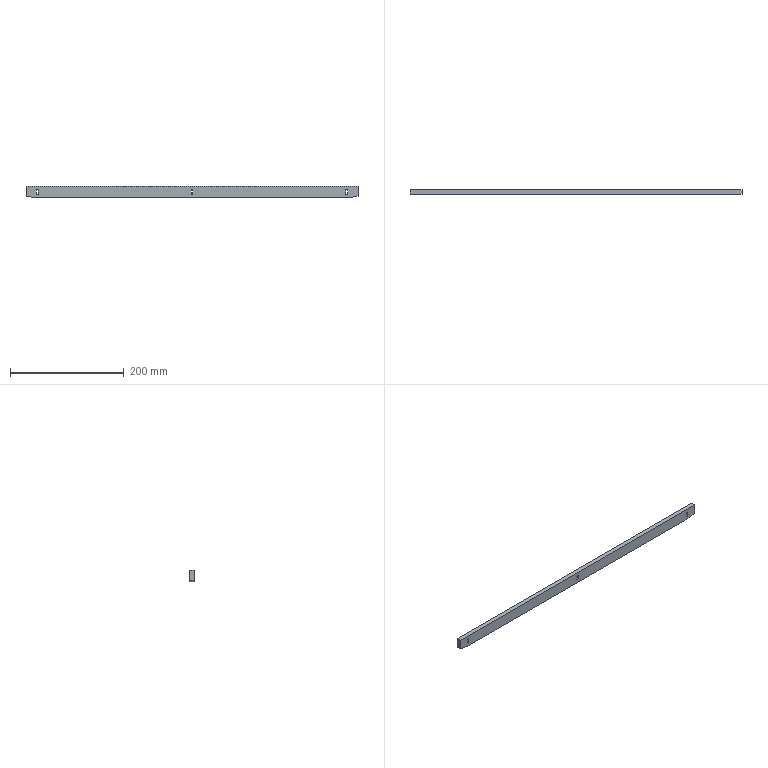Component | SolidWorks | SL010-RightStreamline-1-1_SL010-LXFB-010202-01-1 | 1 solid | 20 faces | box 584 x 8 x 21 mm | volume 97055 mm3 | plane 14 | cylinder 6 | commonest cylinder face diameters 3.2 x6 | material S45C
build123d program:
from build123d import *

# Parameters (mm, degrees)
SKETCH1_W           = 584
SKETCH1_H           = 21
BOSS_EXTRUDE1_DEPTH = 8
CUT_EXTRUDE1_DEPTH  = 293.298
CHAMFER1_SIZE       = 3
CHAMFER1_SIZE2      = 20
CHAMFER2_SIZE       = 20
CHAMFER2_SIZE2      = 3


with BuildPart() as part:
    # Sketch1 → Boss-Extrude1 (new body)
    with BuildSketch(Plane.XY):
        Rectangle(SKETCH1_W, SKETCH1_H)
    extrude(amount=BOSS_EXTRUDE1_DEPTH)

    # Sketch2 → Cut-Extrude1 (cut, through all)
    with BuildSketch(Plane.XY.offset(8)):
        with BuildLine():
            Line((-270.4, 2.5), (-270.4, -2.5))
            ThreePointArc((-270.4, -2.5), (-272, -4.1), (-273.6, -2.5))
            Line((-273.6, -2.5), (-273.6, 2.5))
            ThreePointArc((-273.6, 2.5), (-272, 4.1), (-270.4, 2.5))
        make_face()
        with BuildLine():
            Line((1.6, 2.5), (1.6, -2.5))
            ThreePointArc((1.6, -2.5), (0, -4.1), (-1.6, -2.5))
            Line((-1.6, -2.5), (-1.6, 2.5))
            ThreePointArc((-1.6, 2.5), (0, 4.1), (1.6, 2.5))
        make_face()
        with BuildLine():
            Line((273.6, 2.5), (273.6, -2.5))
            ThreePointArc((273.6, -2.5), (272, -4.1), (270.4, -2.5))
            Line((270.4, -2.5), (270.4, 2.5))
            ThreePointArc((270.4, 2.5), (272, 4.1), (273.6, 2.5))
        make_face()
    extrude(amount=-CUT_EXTRUDE1_DEPTH, mode=Mode.SUBTRACT)

    # Chamfer1
    chamfer1_edges = [part.edges().sort_by_distance(p)[0] for p in [
        (292, 10.5, 4),
    ]]
    chamfer1_side = [part.faces().sort_by_distance(p)[0] for p in [
        (292, 0, 4),
    ]]
    chamfer(chamfer1_edges, length=CHAMFER1_SIZE, length2=CHAMFER1_SIZE2, reference=chamfer1_side[0])

    # Chamfer2
    chamfer2_edges = [part.edges().sort_by_distance(p)[0] for p in [
        (-292, 10.5, 4),
    ]]
    chamfer2_side = [part.faces().sort_by_distance(p)[0] for p in [
        (-10, 10.5, 4),
    ]]
    chamfer(chamfer2_edges, length=CHAMFER2_SIZE, length2=CHAMFER2_SIZE2, reference=chamfer2_side[0])


solid = part.part

# Placed as in the assembly
solid = solid.moved(Location((0, -109.904, -326.535), (-90, 0, 0)))
STEP:
#1=COLOUR_RGB('',0.7922,0.8196,0.9333);
#2=FILL_AREA_STYLE_COLOUR('',#1);
#3=FILL_AREA_STYLE('',(#2));
#4=SURFACE_STYLE_FILL_AREA(#3);
#5=SURFACE_SIDE_STYLE('',(#4));
#6=SURFACE_STYLE_USAGE(.BOTH.,#5);
#7=PRESENTATION_STYLE_ASSIGNMENT((#6));
#8=CARTESIAN_POINT('',(11.496,-4.327,-12.442));
#9=VERTEX_POINT('',#8);
#10=CARTESIAN_POINT('',(11.496,-4.327,-13.151));
#11=VERTEX_POINT('',#10);
#12=CARTESIAN_POINT('',(11.496,-4.327,-13.269));
#13=DIRECTION('',(0.,-0.,-1.));
#14=VECTOR('',#13,39.37);
#15=LINE('',#12,#14);
#16=EDGE_CURVE('',#9,#11,#15,.T.);
#17=ORIENTED_EDGE('',*,*,#16,.T.);
#18=CARTESIAN_POINT('',(11.496,-4.012,-13.151));
#19=VERTEX_POINT('',#18);
#20=CARTESIAN_POINT('',(11.496,-4.012,-13.151));
#21=DIRECTION('',(0.,1.,-0.));
#22=VECTOR('',#21,39.37);
#23=LINE('',#20,#22);
#24=EDGE_CURVE('',#11,#19,#23,.T.);
#25=ORIENTED_EDGE('',*,*,#24,.T.);
#26=CARTESIAN_POINT('',(11.496,-4.012,-12.442));
#27=VERTEX_POINT('',#26);
#28=CARTESIAN_POINT('',(11.496,-4.012,-13.269));
#29=DIRECTION('',(0.,-0.,-1.));
#30=VECTOR('',#29,39.37);
#31=LINE('',#28,#30);
#32=EDGE_CURVE('',#27,#19,#31,.T.);
#33=ORIENTED_EDGE('',*,*,#32,.F.);
#34=CARTESIAN_POINT('',(11.496,-4.012,-12.442));
#35=DIRECTION('',(-0.,-1.,0.));
#36=VECTOR('',#35,39.37);
#37=LINE('',#34,#36);
#38=EDGE_CURVE('',#27,#9,#37,.T.);
#39=ORIENTED_EDGE('',*,*,#38,.T.);
#40=EDGE_LOOP('',(#17,#25,#33,#39));
#41=FACE_OUTER_BOUND('',#40,.T.);
#42=CARTESIAN_POINT('',(11.496,-4.012,-13.269));
#43=DIRECTION('',(-1.,0.,-0.));
#44=DIRECTION('',(0.,1.,-0.));
#45=AXIS2_PLACEMENT_3D('',#42,#43,#44);
#46=PLANE('',#45);
#47=ADVANCED_FACE('',(#41),#46,.F.);
#48=CARTESIAN_POINT('',(10.709,-4.327,-13.269));
#49=VERTEX_POINT('',#48);
#50=CARTESIAN_POINT('',(-10.709,-4.327,-13.269));
#51=VERTEX_POINT('',#50);
#52=CARTESIAN_POINT('',(-11.496,-4.327,-13.269));
#53=DIRECTION('',(-1.,0.,-0.));
#54=VECTOR('',#53,39.37);
#55=LINE('',#52,#54);
#56=EDGE_CURVE('',#49,#51,#55,.T.);
#57=ORIENTED_EDGE('',*,*,#56,.T.);
#58=CARTESIAN_POINT('',(-10.709,-4.012,-13.269));
#59=VERTEX_POINT('',#58);
#60=CARTESIAN_POINT('',(-10.709,-4.012,-13.269));
#61=DIRECTION('',(0.,1.,-0.));
#62=VECTOR('',#61,39.37);
#63=LINE('',#60,#62);
#64=EDGE_CURVE('',#51,#59,#63,.T.);
#65=ORIENTED_EDGE('',*,*,#64,.T.);
#66=CARTESIAN_POINT('',(10.709,-4.012,-13.269));
#67=VERTEX_POINT('',#66);
#68=CARTESIAN_POINT('',(-11.496,-4.012,-13.269));
#69=DIRECTION('',(-1.,0.,-0.));
#70=VECTOR('',#69,39.37);
#71=LINE('',#68,#70);
#72=EDGE_CURVE('',#67,#59,#71,.T.);
#73=ORIENTED_EDGE('',*,*,#72,.F.);
#74=CARTESIAN_POINT('',(10.709,-4.012,-13.269));
#75=DIRECTION('',(-0.,-1.,0.));
#76=VECTOR('',#75,39.37);
#77=LINE('',#74,#76);
#78=EDGE_CURVE('',#67,#49,#77,.T.);
#79=ORIENTED_EDGE('',*,*,#78,.T.);
#80=EDGE_LOOP('',(#57,#65,#73,#79));
#81=FACE_OUTER_BOUND('',#80,.T.);
#82=CARTESIAN_POINT('',(-11.496,-4.012,-13.269));
#83=DIRECTION('',(-0.,0.,1.));
#84=DIRECTION('',(-0.,-1.,0.));
#85=AXIS2_PLACEMENT_3D('',#82,#83,#84);
#86=PLANE('',#85);
#87=ADVANCED_FACE('',(#81),#86,.F.);
#88=CARTESIAN_POINT('',(-11.496,-4.012,-13.151));
#89=VERTEX_POINT('',#88);
#90=CARTESIAN_POINT('',(-11.496,-4.012,-12.442));
#91=VERTEX_POINT('',#90);
#92=CARTESIAN_POINT('',(-11.496,-4.012,-13.269));
#93=DIRECTION('',(-0.,0.,1.));
#94=VECTOR('',#93,39.37);
#95=LINE('',#92,#94);
#96=EDGE_CURVE('',#89,#91,#95,.T.);
#97=ORIENTED_EDGE('',*,*,#96,.F.);
#98=CARTESIAN_POINT('',(-11.496,-4.327,-13.151));
#99=VERTEX_POINT('',#98);
#100=CARTESIAN_POINT('',(-11.496,-4.012,-13.151));
#101=DIRECTION('',(-0.,-1.,0.));
#102=VECTOR('',#101,39.37);
#103=LINE('',#100,#102);
#104=EDGE_CURVE('',#89,#99,#103,.T.);
#105=ORIENTED_EDGE('',*,*,#104,.T.);
#106=CARTESIAN_POINT('',(-11.496,-4.327,-12.442));
#107=VERTEX_POINT('',#106);
#108=CARTESIAN_POINT('',(-11.496,-4.327,-13.269));
#109=DIRECTION('',(-0.,0.,1.));
#110=VECTOR('',#109,39.37);
#111=LINE('',#108,#110);
#112=EDGE_CURVE('',#99,#107,#111,.T.);
#113=ORIENTED_EDGE('',*,*,#112,.T.);
#114=CARTESIAN_POINT('',(-11.496,-4.012,-12.442));
#115=DIRECTION('',(-0.,-1.,0.));
#116=VECTOR('',#115,39.37);
#117=LINE('',#114,#116);
#118=EDGE_CURVE('',#91,#107,#117,.T.);
#119=ORIENTED_EDGE('',*,*,#118,.F.);
#120=EDGE_LOOP('',(#97,#105,#113,#119));
#121=FACE_OUTER_BOUND('',#120,.T.);
#122=CARTESIAN_POINT('',(-11.496,-4.012,-13.269));
#123=DIRECTION('',(1.,-0.,0.));
#124=DIRECTION('',(-0.,-1.,0.));
#125=AXIS2_PLACEMENT_3D('',#122,#123,#124);
#126=PLANE('',#125);
#127=ADVANCED_FACE('',(#121),#126,.F.);
#128=CARTESIAN_POINT('',(-11.496,-4.327,-12.442));
#129=DIRECTION('',(1.,-0.,0.));
#130=VECTOR('',#129,39.37);
#131=LINE('',#128,#130);
#132=EDGE_CURVE('',#107,#9,#131,.T.);
#133=ORIENTED_EDGE('',*,*,#132,.T.);
#134=ORIENTED_EDGE('',*,*,#38,.F.);
#135=CARTESIAN_POINT('',(-11.496,-4.012,-12.442));
#136=DIRECTION('',(1.,-0.,0.));
#137=VECTOR('',#136,39.37);
#138=LINE('',#135,#137);
#139=EDGE_CURVE('',#91,#27,#138,.T.);
#140=ORIENTED_EDGE('',*,*,#139,.F.);
#141=ORIENTED_EDGE('',*,*,#118,.T.);
#142=EDGE_LOOP('',(#133,#134,#140,#141));
#143=FACE_OUTER_BOUND('',#142,.T.);
#144=CARTESIAN_POINT('',(-11.496,-4.012,-12.442));
#145=DIRECTION('',(0.,-0.,-1.));
#146=DIRECTION('',(0.,1.,-0.));
#147=AXIS2_PLACEMENT_3D('',#144,#145,#146);
#148=PLANE('',#147);
#149=ADVANCED_FACE('',(#143),#148,.F.);
#150=CARTESIAN_POINT('',(10.772,-4.012,-12.954));
#151=VERTEX_POINT('',#150);
#152=CARTESIAN_POINT('',(10.646,-4.012,-12.954));
#153=VERTEX_POINT('',#152);
#154=CARTESIAN_POINT('',(10.709,-4.012,-12.954));
#155=DIRECTION('',(0.,1.,-0.));
#156=DIRECTION('',(1.,0.,0.));
#157=AXIS2_PLACEMENT_3D('',#154,#155,#156);
#158=CIRCLE('',#157,0.06299);
#159=EDGE_CURVE('',#151,#153,#158,.T.);
#160=ORIENTED_EDGE('',*,*,#159,.F.);
#161=CARTESIAN_POINT('',(10.772,-4.012,-12.757));
#162=VERTEX_POINT('',#161);
#163=CARTESIAN_POINT('',(10.772,-4.012,-12.954));
#164=DIRECTION('',(0.,-0.,-1.));
#165=VECTOR('',#164,39.37);
#166=LINE('',#163,#165);
#167=EDGE_CURVE('',#162,#151,#166,.T.);
#168=ORIENTED_EDGE('',*,*,#167,.F.);
#169=CARTESIAN_POINT('',(10.646,-4.012,-12.757));
#170=VERTEX_POINT('',#169);
#171=CARTESIAN_POINT('',(10.709,-4.012,-12.757));
#172=DIRECTION('',(0.,1.,-0.));
#173=DIRECTION('',(1.,0.,0.));
#174=AXIS2_PLACEMENT_3D('',#171,#172,#173);
#175=CIRCLE('',#174,0.06299);
#176=EDGE_CURVE('',#170,#162,#175,.T.);
#177=ORIENTED_EDGE('',*,*,#176,.F.);
#178=CARTESIAN_POINT('',(10.646,-4.012,-12.954));
#179=DIRECTION('',(-0.,0.,1.));
#180=VECTOR('',#179,39.37);
#181=LINE('',#178,#180);
#182=EDGE_CURVE('',#153,#170,#181,.T.);
#183=ORIENTED_EDGE('',*,*,#182,.F.);
#184=EDGE_LOOP('',(#160,#168,#177,#183));
#185=FACE_BOUND('',#184,.T.);
#186=CARTESIAN_POINT('',(0.06299,-4.012,-12.954));
#187=VERTEX_POINT('',#186);
#188=CARTESIAN_POINT('',(-0.06299,-4.012,-12.954));
#189=VERTEX_POINT('',#188);
#190=CARTESIAN_POINT('',(-0.,-4.012,-12.954));
#191=DIRECTION('',(0.,1.,-0.));
#192=DIRECTION('',(1.,0.,0.));
#193=AXIS2_PLACEMENT_3D('',#190,#191,#192);
#194=CIRCLE('',#193,0.06299);
#195=EDGE_CURVE('',#187,#189,#194,.T.);
#196=ORIENTED_EDGE('',*,*,#195,.F.);
#197=CARTESIAN_POINT('',(0.06299,-4.012,-12.757));
#198=VERTEX_POINT('',#197);
#199=CARTESIAN_POINT('',(0.06299,-4.012,-12.954));
#200=DIRECTION('',(0.,-0.,-1.));
#201=VECTOR('',#200,39.37);
#202=LINE('',#199,#201);
#203=EDGE_CURVE('',#198,#187,#202,.T.);
#204=ORIENTED_EDGE('',*,*,#203,.F.);
#205=CARTESIAN_POINT('',(-0.06299,-4.012,-12.757));
#206=VERTEX_POINT('',#205);
#207=CARTESIAN_POINT('',(-0.,-4.012,-12.757));
#208=DIRECTION('',(0.,1.,-0.));
#209=DIRECTION('',(1.,0.,0.));
#210=AXIS2_PLACEMENT_3D('',#207,#208,#209);
#211=CIRCLE('',#210,0.06299);
#212=EDGE_CURVE('',#206,#198,#211,.T.);
#213=ORIENTED_EDGE('',*,*,#212,.F.);
#214=CARTESIAN_POINT('',(-0.06299,-4.012,-12.954));
#215=DIRECTION('',(-0.,0.,1.));
#216=VECTOR('',#215,39.37);
#217=LINE('',#214,#216);
#218=EDGE_CURVE('',#189,#206,#217,.T.);
#219=ORIENTED_EDGE('',*,*,#218,.F.);
#220=EDGE_LOOP('',(#196,#204,#213,#219));
#221=FACE_BOUND('',#220,.T.);
#222=CARTESIAN_POINT('',(-10.646,-4.012,-12.954));
#223=VERTEX_POINT('',#222);
#224=CARTESIAN_POINT('',(-10.772,-4.012,-12.954));
#225=VERTEX_POINT('',#224);
#226=CARTESIAN_POINT('',(-10.709,-4.012,-12.954));
#227=DIRECTION('',(0.,1.,-0.));
#228=DIRECTION('',(1.,0.,0.));
#229=AXIS2_PLACEMENT_3D('',#226,#227,#228);
#230=CIRCLE('',#229,0.06299);
#231=EDGE_CURVE('',#223,#225,#230,.T.);
#232=ORIENTED_EDGE('',*,*,#231,.F.);
#233=CARTESIAN_POINT('',(-10.646,-4.012,-12.757));
#234=VERTEX_POINT('',#233);
#235=CARTESIAN_POINT('',(-10.646,-4.012,-12.954));
#236=DIRECTION('',(0.,-0.,-1.));
#237=VECTOR('',#236,39.37);
#238=LINE('',#235,#237);
#239=EDGE_CURVE('',#234,#223,#238,.T.);
#240=ORIENTED_EDGE('',*,*,#239,.F.);
#241=CARTESIAN_POINT('',(-10.772,-4.012,-12.757));
#242=VERTEX_POINT('',#241);
#243=CARTESIAN_POINT('',(-10.709,-4.012,-12.757));
#244=DIRECTION('',(0.,1.,-0.));
#245=DIRECTION('',(1.,0.,0.));
#246=AXIS2_PLACEMENT_3D('',#243,#244,#245);
#247=CIRCLE('',#246,0.06299);
#248=EDGE_CURVE('',#242,#234,#247,.T.);
#249=ORIENTED_EDGE('',*,*,#248,.F.);
#250=CARTESIAN_POINT('',(-10.772,-4.012,-12.954));
#251=DIRECTION('',(-0.,0.,1.));
#252=VECTOR('',#251,39.37);
#253=LINE('',#250,#252);
#254=EDGE_CURVE('',#225,#242,#253,.T.);
#255=ORIENTED_EDGE('',*,*,#254,.F.);
#256=EDGE_LOOP('',(#232,#240,#249,#255));
#257=FACE_BOUND('',#256,.T.);
#258=ORIENTED_EDGE('',*,*,#72,.T.);
#259=CARTESIAN_POINT('',(-0.2963,-4.012,-14.831));
#260=DIRECTION('',(-0.9889,0.,0.1483));
#261=VECTOR('',#260,39.37);
#262=LINE('',#259,#261);
#263=EDGE_CURVE('',#59,#89,#262,.T.);
#264=ORIENTED_EDGE('',*,*,#263,.T.);
#265=ORIENTED_EDGE('',*,*,#96,.T.);
#266=ORIENTED_EDGE('',*,*,#139,.T.);
#267=ORIENTED_EDGE('',*,*,#32,.T.);
#268=CARTESIAN_POINT('',(0.2963,-4.012,-14.831));
#269=DIRECTION('',(-0.9889,0.,-0.1483));
#270=VECTOR('',#269,39.37);
#271=LINE('',#268,#270);
#272=EDGE_CURVE('',#19,#67,#271,.T.);
#273=ORIENTED_EDGE('',*,*,#272,.T.);
#274=EDGE_LOOP('',(#258,#264,#265,#266,#267,#273));
#275=FACE_OUTER_BOUND('',#274,.T.);
#276=CARTESIAN_POINT('',(-0.,-4.012,-12.856));
#277=DIRECTION('',(0.,1.,-0.));
#278=DIRECTION('',(1.,-0.,0.));
#279=AXIS2_PLACEMENT_3D('',#276,#277,#278);
#280=PLANE('',#279);
#281=ADVANCED_FACE('',(#185,#221,#257,#275),#280,.T.);
#282=CARTESIAN_POINT('',(10.772,-4.327,-12.757));
#283=VERTEX_POINT('',#282);
#284=CARTESIAN_POINT('',(10.772,-4.327,-12.954));
#285=VERTEX_POINT('',#284);
#286=CARTESIAN_POINT('',(10.772,-4.327,-12.954));
#287=DIRECTION('',(0.,-0.,-1.));
#288=VECTOR('',#287,39.37);
#289=LINE('',#286,#288);
#290=EDGE_CURVE('',#283,#285,#289,.T.);
#291=ORIENTED_EDGE('',*,*,#290,.T.);
#292=CARTESIAN_POINT('',(10.646,-4.327,-12.954));
#293=VERTEX_POINT('',#292);
#294=CARTESIAN_POINT('',(10.709,-4.327,-12.954));
#295=DIRECTION('',(0.,1.,-0.));
#296=DIRECTION('',(1.,0.,0.));
#297=AXIS2_PLACEMENT_3D('',#294,#295,#296);
#298=CIRCLE('',#297,0.06299);
#299=EDGE_CURVE('',#285,#293,#298,.T.);
#300=ORIENTED_EDGE('',*,*,#299,.T.);
#301=CARTESIAN_POINT('',(10.646,-4.327,-12.757));
#302=VERTEX_POINT('',#301);
#303=CARTESIAN_POINT('',(10.646,-4.327,-12.954));
#304=DIRECTION('',(-0.,0.,1.));
#305=VECTOR('',#304,39.37);
#306=LINE('',#303,#305);
#307=EDGE_CURVE('',#293,#302,#306,.T.);
#308=ORIENTED_EDGE('',*,*,#307,.T.);
#309=CARTESIAN_POINT('',(10.709,-4.327,-12.757));
#310=DIRECTION('',(0.,1.,-0.));
#311=DIRECTION('',(1.,0.,0.));
#312=AXIS2_PLACEMENT_3D('',#309,#310,#311);
#313=CIRCLE('',#312,0.06299);
#314=EDGE_CURVE('',#302,#283,#313,.T.);
#315=ORIENTED_EDGE('',*,*,#314,.T.);
#316=EDGE_LOOP('',(#291,#300,#308,#315));
#317=FACE_BOUND('',#316,.T.);
#318=CARTESIAN_POINT('',(0.06299,-4.327,-12.757));
#319=VERTEX_POINT('',#318);
#320=CARTESIAN_POINT('',(0.06299,-4.327,-12.954));
#321=VERTEX_POINT('',#320);
#322=CARTESIAN_POINT('',(0.06299,-4.327,-12.954));
#323=DIRECTION('',(0.,-0.,-1.));
#324=VECTOR('',#323,39.37);
#325=LINE('',#322,#324);
#326=EDGE_CURVE('',#319,#321,#325,.T.);
#327=ORIENTED_EDGE('',*,*,#326,.T.);
#328=CARTESIAN_POINT('',(-0.06299,-4.327,-12.954));
#329=VERTEX_POINT('',#328);
#330=CARTESIAN_POINT('',(-0.,-4.327,-12.954));
#331=DIRECTION('',(0.,1.,-0.));
#332=DIRECTION('',(1.,0.,0.));
#333=AXIS2_PLACEMENT_3D('',#330,#331,#332);
#334=CIRCLE('',#333,0.06299);
#335=EDGE_CURVE('',#321,#329,#334,.T.);
#336=ORIENTED_EDGE('',*,*,#335,.T.);
#337=CARTESIAN_POINT('',(-0.06299,-4.327,-12.757));
#338=VERTEX_POINT('',#337);
#339=CARTESIAN_POINT('',(-0.06299,-4.327,-12.954));
#340=DIRECTION('',(-0.,0.,1.));
#341=VECTOR('',#340,39.37);
#342=LINE('',#339,#341);
#343=EDGE_CURVE('',#329,#338,#342,.T.);
#344=ORIENTED_EDGE('',*,*,#343,.T.);
#345=CARTESIAN_POINT('',(-0.,-4.327,-12.757));
#346=DIRECTION('',(0.,1.,-0.));
#347=DIRECTION('',(1.,0.,0.));
#348=AXIS2_PLACEMENT_3D('',#345,#346,#347);
#349=CIRCLE('',#348,0.06299);
#350=EDGE_CURVE('',#338,#319,#349,.T.);
#351=ORIENTED_EDGE('',*,*,#350,.T.);
#352=EDGE_LOOP('',(#327,#336,#344,#351));
#353=FACE_BOUND('',#352,.T.);
#354=CARTESIAN_POINT('',(-10.646,-4.327,-12.757));
#355=VERTEX_POINT('',#354);
#356=CARTESIAN_POINT('',(-10.646,-4.327,-12.954));
#357=VERTEX_POINT('',#356);
#358=CARTESIAN_POINT('',(-10.646,-4.327,-12.954));
#359=DIRECTION('',(0.,-0.,-1.));
#360=VECTOR('',#359,39.37);
#361=LINE('',#358,#360);
#362=EDGE_CURVE('',#355,#357,#361,.T.);
#363=ORIENTED_EDGE('',*,*,#362,.T.);
#364=CARTESIAN_POINT('',(-10.772,-4.327,-12.954));
#365=VERTEX_POINT('',#364);
#366=CARTESIAN_POINT('',(-10.709,-4.327,-12.954));
#367=DIRECTION('',(0.,1.,-0.));
#368=DIRECTION('',(1.,0.,0.));
#369=AXIS2_PLACEMENT_3D('',#366,#367,#368);
#370=CIRCLE('',#369,0.06299);
#371=EDGE_CURVE('',#357,#365,#370,.T.);
#372=ORIENTED_EDGE('',*,*,#371,.T.);
#373=CARTESIAN_POINT('',(-10.772,-4.327,-12.757));
#374=VERTEX_POINT('',#373);
#375=CARTESIAN_POINT('',(-10.772,-4.327,-12.954));
#376=DIRECTION('',(-0.,0.,1.));
#377=VECTOR('',#376,39.37);
#378=LINE('',#375,#377);
#379=EDGE_CURVE('',#365,#374,#378,.T.);
#380=ORIENTED_EDGE('',*,*,#379,.T.);
#381=CARTESIAN_POINT('',(-10.709,-4.327,-12.757));
#382=DIRECTION('',(0.,1.,-0.));
#383=DIRECTION('',(1.,0.,0.));
#384=AXIS2_PLACEMENT_3D('',#381,#382,#383);
#385=CIRCLE('',#384,0.06299);
#386=EDGE_CURVE('',#374,#355,#385,.T.);
#387=ORIENTED_EDGE('',*,*,#386,.T.);
#388=EDGE_LOOP('',(#363,#372,#380,#387));
#389=FACE_BOUND('',#388,.T.);
#390=ORIENTED_EDGE('',*,*,#112,.F.);
#391=CARTESIAN_POINT('',(-11.496,-4.327,-13.151));
#392=DIRECTION('',(0.9889,-0.,-0.1483));
#393=VECTOR('',#392,39.37);
#394=LINE('',#391,#393);
#395=EDGE_CURVE('',#99,#51,#394,.T.);
#396=ORIENTED_EDGE('',*,*,#395,.T.);
#397=ORIENTED_EDGE('',*,*,#56,.F.);
#398=CARTESIAN_POINT('',(10.709,-4.327,-13.269));
#399=DIRECTION('',(0.9889,-0.,0.1483));
#400=VECTOR('',#399,39.37);
#401=LINE('',#398,#400);
#402=EDGE_CURVE('',#49,#11,#401,.T.);
#403=ORIENTED_EDGE('',*,*,#402,.T.);
#404=ORIENTED_EDGE('',*,*,#16,.F.);
#405=ORIENTED_EDGE('',*,*,#132,.F.);
#406=EDGE_LOOP('',(#390,#396,#397,#403,#404,#405));
#407=FACE_OUTER_BOUND('',#406,.T.);
#408=CARTESIAN_POINT('',(-0.,-4.327,-12.856));
#409=DIRECTION('',(0.,1.,-0.));
#410=DIRECTION('',(1.,-0.,0.));
#411=AXIS2_PLACEMENT_3D('',#408,#409,#410);
#412=PLANE('',#411);
#413=ADVANCED_FACE('',(#317,#353,#389,#407),#412,.F.);
#414=ORIENTED_EDGE('',*,*,#231,.T.);
#415=CARTESIAN_POINT('',(-10.772,-4.327,-12.954));
#416=DIRECTION('',(0.,1.,-0.));
#417=VECTOR('',#416,39.37);
#418=LINE('',#415,#417);
#419=EDGE_CURVE('',#365,#225,#418,.T.);
#420=ORIENTED_EDGE('',*,*,#419,.F.);
#421=ORIENTED_EDGE('',*,*,#371,.F.);
#422=CARTESIAN_POINT('',(-10.646,-4.327,-12.954));
#423=DIRECTION('',(0.,1.,-0.));
#424=VECTOR('',#423,39.37);
#425=LINE('',#422,#424);
#426=EDGE_CURVE('',#357,#223,#425,.T.);
#427=ORIENTED_EDGE('',*,*,#426,.T.);
#428=EDGE_LOOP('',(#414,#420,#421,#427));
#429=FACE_OUTER_BOUND('',#428,.T.);
#430=CARTESIAN_POINT('',(-10.709,-4.327,-12.954));
#431=DIRECTION('',(0.,1.,-0.));
#432=DIRECTION('',(1.,0.,0.));
#433=AXIS2_PLACEMENT_3D('',#430,#431,#432);
#434=CYLINDRICAL_SURFACE('',#433,0.06299);
#435=ADVANCED_FACE('',(#429),#434,.F.);
#436=ORIENTED_EDGE('',*,*,#239,.T.);
#437=ORIENTED_EDGE('',*,*,#426,.F.);
#438=ORIENTED_EDGE('',*,*,#362,.F.);
#439=CARTESIAN_POINT('',(-10.646,-4.327,-12.757));
#440=DIRECTION('',(0.,1.,-0.));
#441=VECTOR('',#440,39.37);
#442=LINE('',#439,#441);
#443=EDGE_CURVE('',#355,#234,#442,.T.);
#444=ORIENTED_EDGE('',*,*,#443,.T.);
#445=EDGE_LOOP('',(#436,#437,#438,#444));
#446=FACE_OUTER_BOUND('',#445,.T.);
#447=CARTESIAN_POINT('',(-10.646,-4.327,-12.954));
#448=DIRECTION('',(1.,-0.,0.));
#449=DIRECTION('',(-0.,-1.,0.));
#450=AXIS2_PLACEMENT_3D('',#447,#448,#449);
#451=PLANE('',#450);
#452=ADVANCED_FACE('',(#446),#451,.F.);
#453=ORIENTED_EDGE('',*,*,#248,.T.);
#454=ORIENTED_EDGE('',*,*,#443,.F.);
#455=ORIENTED_EDGE('',*,*,#386,.F.);
#456=CARTESIAN_POINT('',(-10.772,-4.327,-12.757));
#457=DIRECTION('',(0.,1.,-0.));
#458=VECTOR('',#457,39.37);
#459=LINE('',#456,#458);
#460=EDGE_CURVE('',#374,#242,#459,.T.);
#461=ORIENTED_EDGE('',*,*,#460,.T.);
#462=EDGE_LOOP('',(#453,#454,#455,#461));
#463=FACE_OUTER_BOUND('',#462,.T.);
#464=CARTESIAN_POINT('',(-10.709,-4.327,-12.757));
#465=DIRECTION('',(0.,1.,-0.));
#466=DIRECTION('',(1.,0.,0.));
#467=AXIS2_PLACEMENT_3D('',#464,#465,#466);
#468=CYLINDRICAL_SURFACE('',#467,0.06299);
#469=ADVANCED_FACE('',(#463),#468,.F.);
#470=ORIENTED_EDGE('',*,*,#254,.T.);
#471=ORIENTED_EDGE('',*,*,#460,.F.);
#472=ORIENTED_EDGE('',*,*,#379,.F.);
#473=ORIENTED_EDGE('',*,*,#419,.T.);
#474=EDGE_LOOP('',(#470,#471,#472,#473));
#475=FACE_OUTER_BOUND('',#474,.T.);
#476=CARTESIAN_POINT('',(-10.772,-4.327,-12.954));
#477=DIRECTION('',(-1.,0.,-0.));
#478=DIRECTION('',(0.,1.,-0.));
#479=AXIS2_PLACEMENT_3D('',#476,#477,#478);
#480=PLANE('',#479);
#481=ADVANCED_FACE('',(#475),#480,.F.);
#482=ORIENTED_EDGE('',*,*,#195,.T.);
#483=CARTESIAN_POINT('',(-0.06299,-4.327,-12.954));
#484=DIRECTION('',(0.,1.,-0.));
#485=VECTOR('',#484,39.37);
#486=LINE('',#483,#485);
#487=EDGE_CURVE('',#329,#189,#486,.T.);
#488=ORIENTED_EDGE('',*,*,#487,.F.);
#489=ORIENTED_EDGE('',*,*,#335,.F.);
#490=CARTESIAN_POINT('',(0.06299,-4.327,-12.954));
#491=DIRECTION('',(0.,1.,-0.));
#492=VECTOR('',#491,39.37);
#493=LINE('',#490,#492);
#494=EDGE_CURVE('',#321,#187,#493,.T.);
#495=ORIENTED_EDGE('',*,*,#494,.T.);
#496=EDGE_LOOP('',(#482,#488,#489,#495));
#497=FACE_OUTER_BOUND('',#496,.T.);
#498=CARTESIAN_POINT('',(-0.,-4.327,-12.954));
#499=DIRECTION('',(0.,1.,-0.));
#500=DIRECTION('',(1.,0.,0.));
#501=AXIS2_PLACEMENT_3D('',#498,#499,#500);
#502=CYLINDRICAL_SURFACE('',#501,0.06299);
#503=ADVANCED_FACE('',(#497),#502,.F.);
#504=ORIENTED_EDGE('',*,*,#203,.T.);
#505=ORIENTED_EDGE('',*,*,#494,.F.);
#506=ORIENTED_EDGE('',*,*,#326,.F.);
#507=CARTESIAN_POINT('',(0.06299,-4.327,-12.757));
#508=DIRECTION('',(0.,1.,-0.));
#509=VECTOR('',#508,39.37);
#510=LINE('',#507,#509);
#511=EDGE_CURVE('',#319,#198,#510,.T.);
#512=ORIENTED_EDGE('',*,*,#511,.T.);
#513=EDGE_LOOP('',(#504,#505,#506,#512));
#514=FACE_OUTER_BOUND('',#513,.T.);
#515=CARTESIAN_POINT('',(0.06299,-4.327,-12.954));
#516=DIRECTION('',(1.,-0.,0.));
#517=DIRECTION('',(-0.,-1.,0.));
#518=AXIS2_PLACEMENT_3D('',#515,#516,#517);
#519=PLANE('',#518);
#520=ADVANCED_FACE('',(#514),#519,.F.);
#521=ORIENTED_EDGE('',*,*,#212,.T.);
#522=ORIENTED_EDGE('',*,*,#511,.F.);
#523=ORIENTED_EDGE('',*,*,#350,.F.);
#524=CARTESIAN_POINT('',(-0.06299,-4.327,-12.757));
#525=DIRECTION('',(0.,1.,-0.));
#526=VECTOR('',#525,39.37);
#527=LINE('',#524,#526);
#528=EDGE_CURVE('',#338,#206,#527,.T.);
#529=ORIENTED_EDGE('',*,*,#528,.T.);
#530=EDGE_LOOP('',(#521,#522,#523,#529));
#531=FACE_OUTER_BOUND('',#530,.T.);
#532=CARTESIAN_POINT('',(-0.,-4.327,-12.757));
#533=DIRECTION('',(0.,1.,-0.));
#534=DIRECTION('',(1.,0.,0.));
#535=AXIS2_PLACEMENT_3D('',#532,#533,#534);
#536=CYLINDRICAL_SURFACE('',#535,0.06299);
#537=ADVANCED_FACE('',(#531),#536,.F.);
#538=ORIENTED_EDGE('',*,*,#218,.T.);
#539=ORIENTED_EDGE('',*,*,#528,.F.);
#540=ORIENTED_EDGE('',*,*,#343,.F.);
#541=ORIENTED_EDGE('',*,*,#487,.T.);
#542=EDGE_LOOP('',(#538,#539,#540,#541));
#543=FACE_OUTER_BOUND('',#542,.T.);
#544=CARTESIAN_POINT('',(-0.06299,-4.327,-12.954));
#545=DIRECTION('',(-1.,0.,-0.));
#546=DIRECTION('',(0.,1.,-0.));
#547=AXIS2_PLACEMENT_3D('',#544,#545,#546);
#548=PLANE('',#547);
#549=ADVANCED_FACE('',(#543),#548,.F.);
#550=ORIENTED_EDGE('',*,*,#159,.T.);
#551=CARTESIAN_POINT('',(10.646,-4.327,-12.954));
#552=DIRECTION('',(0.,1.,-0.));
#553=VECTOR('',#552,39.37);
#554=LINE('',#551,#553);
#555=EDGE_CURVE('',#293,#153,#554,.T.);
#556=ORIENTED_EDGE('',*,*,#555,.F.);
#557=ORIENTED_EDGE('',*,*,#299,.F.);
#558=CARTESIAN_POINT('',(10.772,-4.327,-12.954));
#559=DIRECTION('',(0.,1.,-0.));
#560=VECTOR('',#559,39.37);
#561=LINE('',#558,#560);
#562=EDGE_CURVE('',#285,#151,#561,.T.);
#563=ORIENTED_EDGE('',*,*,#562,.T.);
#564=EDGE_LOOP('',(#550,#556,#557,#563));
#565=FACE_OUTER_BOUND('',#564,.T.);
#566=CARTESIAN_POINT('',(10.709,-4.327,-12.954));
#567=DIRECTION('',(0.,1.,-0.));
#568=DIRECTION('',(1.,0.,0.));
#569=AXIS2_PLACEMENT_3D('',#566,#567,#568);
#570=CYLINDRICAL_SURFACE('',#569,0.06299);
#571=ADVANCED_FACE('',(#565),#570,.F.);
#572=ORIENTED_EDGE('',*,*,#167,.T.);
#573=ORIENTED_EDGE('',*,*,#562,.F.);
#574=ORIENTED_EDGE('',*,*,#290,.F.);
#575=CARTESIAN_POINT('',(10.772,-4.327,-12.757));
#576=DIRECTION('',(0.,1.,-0.));
#577=VECTOR('',#576,39.37);
#578=LINE('',#575,#577);
#579=EDGE_CURVE('',#283,#162,#578,.T.);
#580=ORIENTED_EDGE('',*,*,#579,.T.);
#581=EDGE_LOOP('',(#572,#573,#574,#580));
#582=FACE_OUTER_BOUND('',#581,.T.);
#583=CARTESIAN_POINT('',(10.772,-4.327,-12.954));
#584=DIRECTION('',(1.,-0.,0.));
#585=DIRECTION('',(-0.,-1.,0.));
#586=AXIS2_PLACEMENT_3D('',#583,#584,#585);
#587=PLANE('',#586);
#588=ADVANCED_FACE('',(#582),#587,.F.);
#589=ORIENTED_EDGE('',*,*,#176,.T.);
#590=ORIENTED_EDGE('',*,*,#579,.F.);
#591=ORIENTED_EDGE('',*,*,#314,.F.);
#592=CARTESIAN_POINT('',(10.646,-4.327,-12.757));
#593=DIRECTION('',(0.,1.,-0.));
#594=VECTOR('',#593,39.37);
#595=LINE('',#592,#594);
#596=EDGE_CURVE('',#302,#170,#595,.T.);
#597=ORIENTED_EDGE('',*,*,#596,.T.);
#598=EDGE_LOOP('',(#589,#590,#591,#597));
#599=FACE_OUTER_BOUND('',#598,.T.);
#600=CARTESIAN_POINT('',(10.709,-4.327,-12.757));
#601=DIRECTION('',(0.,1.,-0.));
#602=DIRECTION('',(1.,0.,0.));
#603=AXIS2_PLACEMENT_3D('',#600,#601,#602);
#604=CYLINDRICAL_SURFACE('',#603,0.06299);
#605=ADVANCED_FACE('',(#599),#604,.F.);
#606=ORIENTED_EDGE('',*,*,#182,.T.);
#607=ORIENTED_EDGE('',*,*,#596,.F.);
#608=ORIENTED_EDGE('',*,*,#307,.F.);
#609=ORIENTED_EDGE('',*,*,#555,.T.);
#610=EDGE_LOOP('',(#606,#607,#608,#609));
#611=FACE_OUTER_BOUND('',#610,.T.);
#612=CARTESIAN_POINT('',(10.646,-4.327,-12.954));
#613=DIRECTION('',(-1.,0.,-0.));
#614=DIRECTION('',(0.,1.,-0.));
#615=AXIS2_PLACEMENT_3D('',#612,#613,#614);
#616=PLANE('',#615);
#617=ADVANCED_FACE('',(#611),#616,.F.);
#618=ORIENTED_EDGE('',*,*,#272,.F.);
#619=ORIENTED_EDGE('',*,*,#24,.F.);
#620=ORIENTED_EDGE('',*,*,#402,.F.);
#621=ORIENTED_EDGE('',*,*,#78,.F.);
#622=EDGE_LOOP('',(#618,#619,#620,#621));
#623=FACE_OUTER_BOUND('',#622,.T.);
#624=CARTESIAN_POINT('',(10.709,-4.012,-13.269));
#625=DIRECTION('',(-0.1483,0.,0.9889));
#626=DIRECTION('',(-0.,-1.,0.));
#627=AXIS2_PLACEMENT_3D('',#624,#625,#626);
#628=PLANE('',#627);
#629=ADVANCED_FACE('',(#623),#628,.F.);
#630=ORIENTED_EDGE('',*,*,#263,.F.);
#631=ORIENTED_EDGE('',*,*,#64,.F.);
#632=ORIENTED_EDGE('',*,*,#395,.F.);
#633=ORIENTED_EDGE('',*,*,#104,.F.);
#634=EDGE_LOOP('',(#630,#631,#632,#633));
#635=FACE_OUTER_BOUND('',#634,.T.);
#636=CARTESIAN_POINT('',(-11.496,-4.012,-13.151));
#637=DIRECTION('',(0.1483,0.,0.9889));
#638=DIRECTION('',(-0.,-1.,0.));
#639=AXIS2_PLACEMENT_3D('',#636,#637,#638);
#640=PLANE('',#639);
#641=ADVANCED_FACE('',(#635),#640,.F.);
#642=CLOSED_SHELL('',(#47,#87,#127,#149,#281,#413,#435,#452,#469,#481,#503,#520,#537,#549,#571,#588,#605,#617,#629,#641));
#643=MANIFOLD_SOLID_BREP('',#642);
#644=STYLED_ITEM('',(#7),#643);
#645=(LENGTH_UNIT()NAMED_UNIT(*)SI_UNIT($,.METRE.));
#646=LENGTH_MEASURE_WITH_UNIT(LENGTH_MEASURE(0.0254),#645);
#647=DIMENSIONAL_EXPONENTS(1.,0.,0.,0.,0.,0.,0.);
#648=(CONVERSION_BASED_UNIT('',#646)LENGTH_UNIT()NAMED_UNIT(#647));
#649=UNCERTAINTY_MEASURE_WITH_UNIT(LENGTH_MEASURE(0.00001),#648,'','');
#650=(NAMED_UNIT(*)PLANE_ANGLE_UNIT()SI_UNIT($,.RADIAN.));
#651=(NAMED_UNIT(*)SI_UNIT($,.STERADIAN.)SOLID_ANGLE_UNIT());
#652=(GEOMETRIC_REPRESENTATION_CONTEXT(3)GLOBAL_UNCERTAINTY_ASSIGNED_CONTEXT((#649))GLOBAL_UNIT_ASSIGNED_CONTEXT((#648,#650,#651))REPRESENTATION_CONTEXT('',''));
#653=MECHANICAL_DESIGN_GEOMETRIC_PRESENTATION_REPRESENTATION('',(#644),#652);
#654=CARTESIAN_POINT('',(0.,0.,0.));
#655=DIRECTION('',(0.,0.,1.));
#656=DIRECTION('',(1.,0.,0.));
#657=AXIS2_PLACEMENT_3D('',#654,#655,#656);
#658=(LENGTH_UNIT()NAMED_UNIT(*)SI_UNIT($,.METRE.));
#659=LENGTH_MEASURE_WITH_UNIT(LENGTH_MEASURE(0.0254),#658);
#660=DIMENSIONAL_EXPONENTS(1.,0.,0.,0.,0.,0.,0.);
#661=(CONVERSION_BASED_UNIT('',#659)LENGTH_UNIT()NAMED_UNIT(#660));
#662=UNCERTAINTY_MEASURE_WITH_UNIT(LENGTH_MEASURE(0.00001),#661,'','');
#663=(NAMED_UNIT(*)PLANE_ANGLE_UNIT()SI_UNIT($,.RADIAN.));
#664=(NAMED_UNIT(*)SI_UNIT($,.STERADIAN.)SOLID_ANGLE_UNIT());
#665=(GEOMETRIC_REPRESENTATION_CONTEXT(3)GLOBAL_UNCERTAINTY_ASSIGNED_CONTEXT((#662))GLOBAL_UNIT_ASSIGNED_CONTEXT((#661,#663,#664))REPRESENTATION_CONTEXT('',''));
#666=ADVANCED_BREP_SHAPE_REPRESENTATION('',(#643,#657),#665);
#667=PRESENTATION_LAYER_ASSIGNMENT('','',(#644));